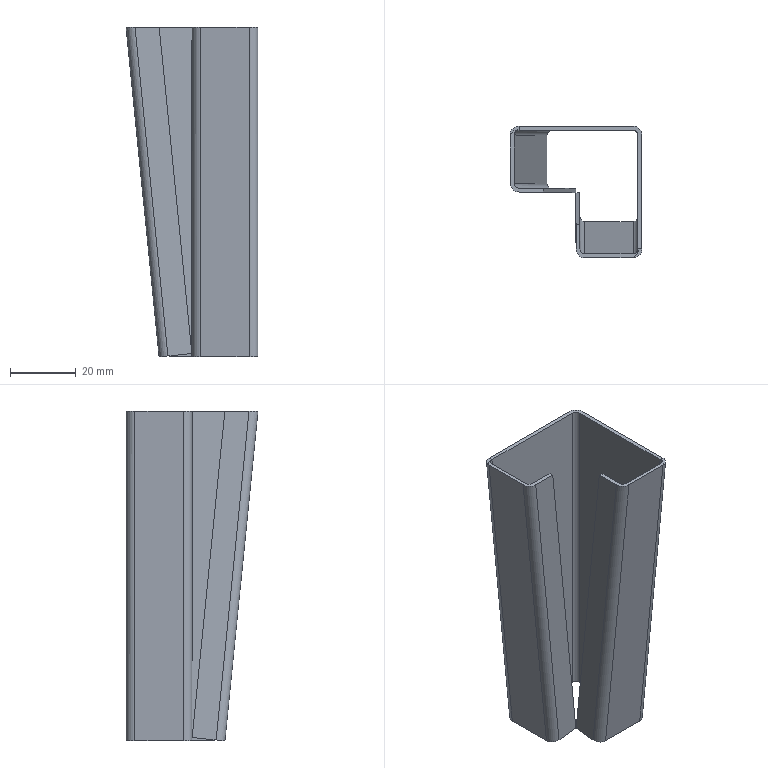Component | SolidWorks | Seat-1 | 1 solid | 42 faces | volume 14354 mm3 | plane 30 | cylinder 10 | spline 2 | commonest cylinder face diameters 5.4 x5 3 x5